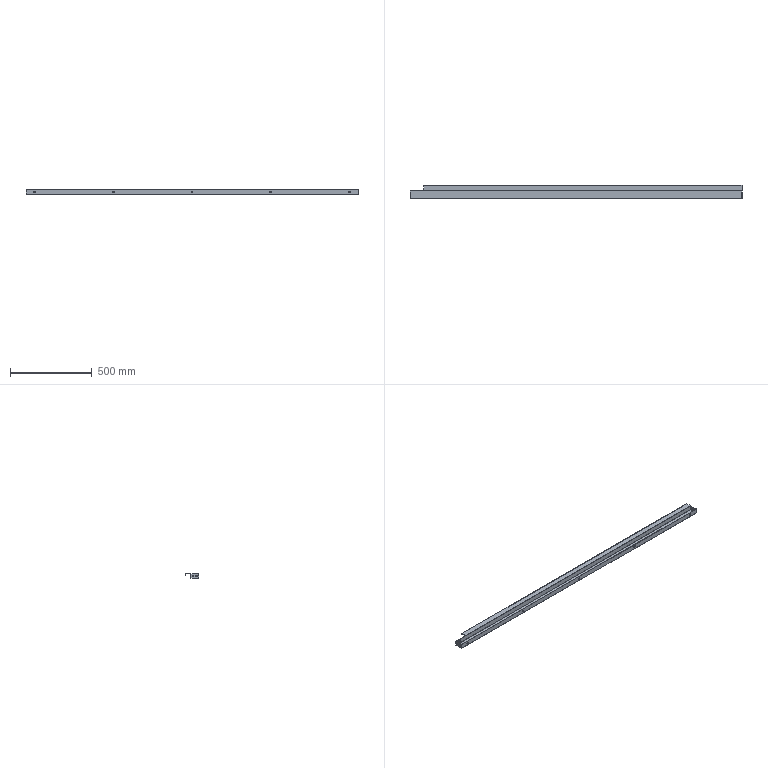Component | SolidWorks | LowerCrossbeam20001234-1 | 1 solid | 84 faces | volume 442422 mm3 | plane 50 | cylinder 34 | commonest cylinder face diameters 11 x14 9 x8 3.4 x5 0.4 x5 7 x1 4 x1